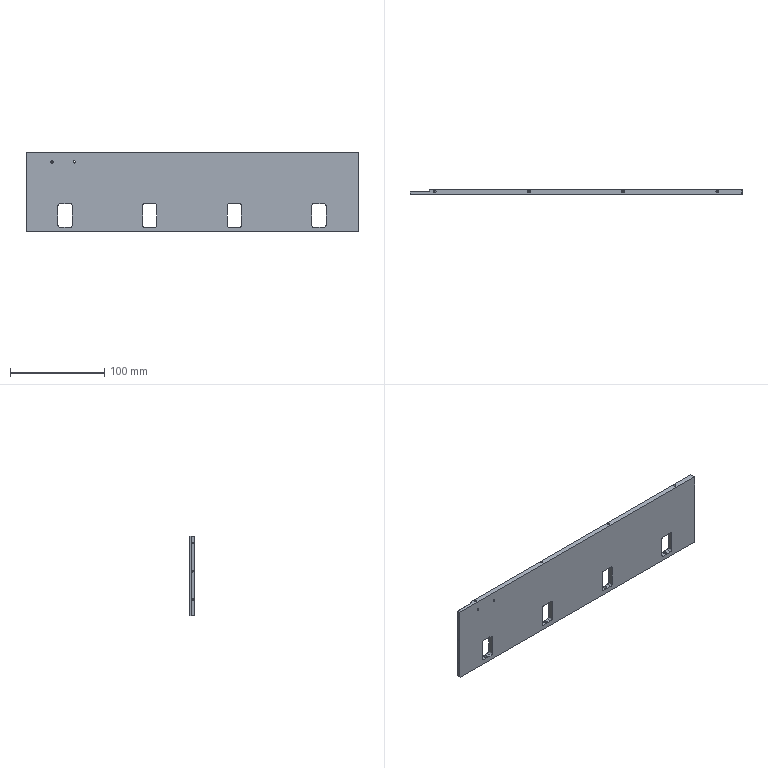CAM job | Mastercam | mm | 9 operations | part box 353 x 5.5 x 85
1. Drill/Counterbore | 2 - 6定位倒角
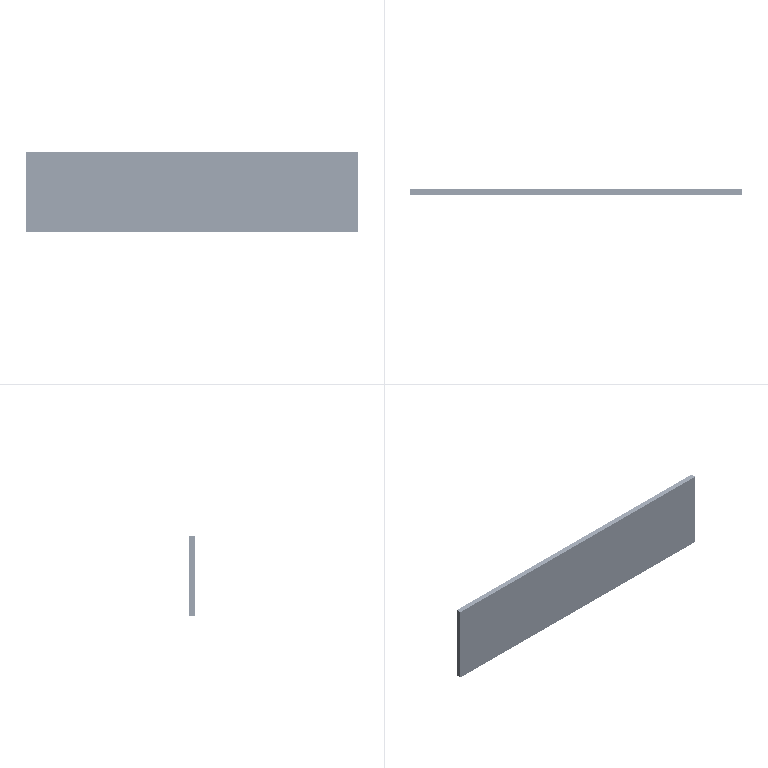2. Peck Drill | 18 - 3.6 钻头
3. Drill/Counterbore | 2 - 6定位倒角
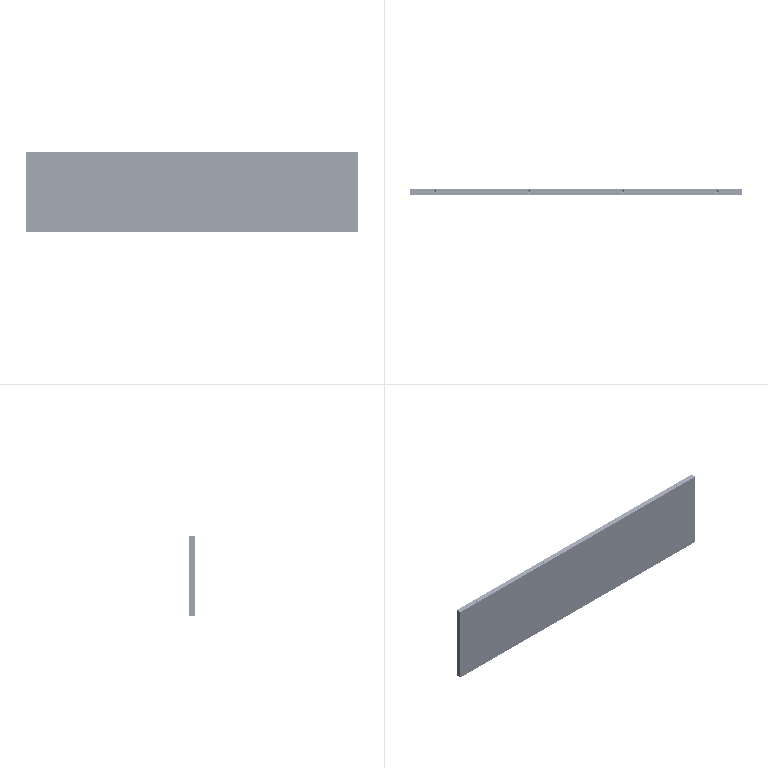4. Peck Drill | 12 - 2.5 钻头
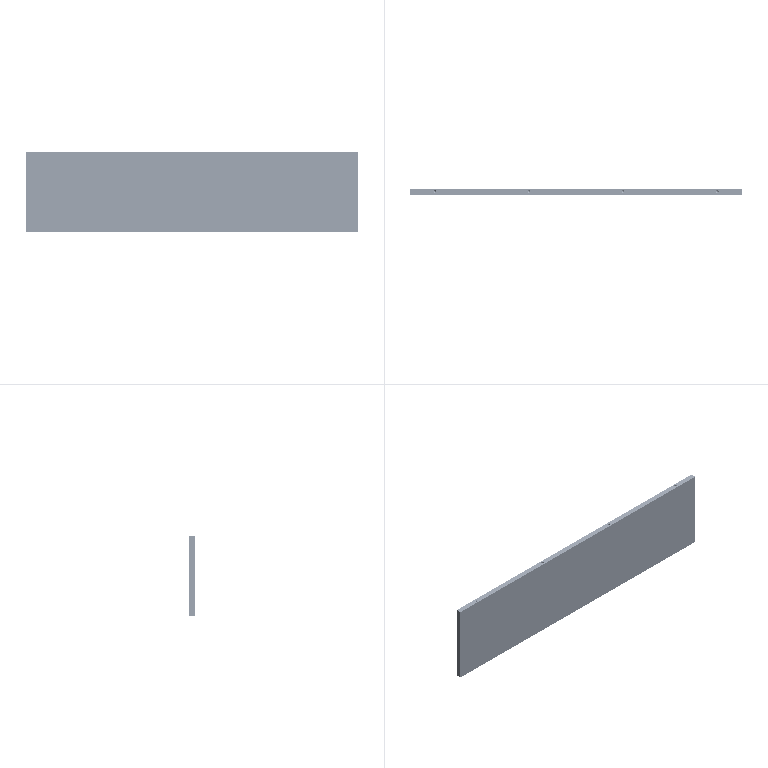5. Peck Drill | 12 - 2.5 钻头
6. Drill/Counterbore | 2 - 6定位倒角
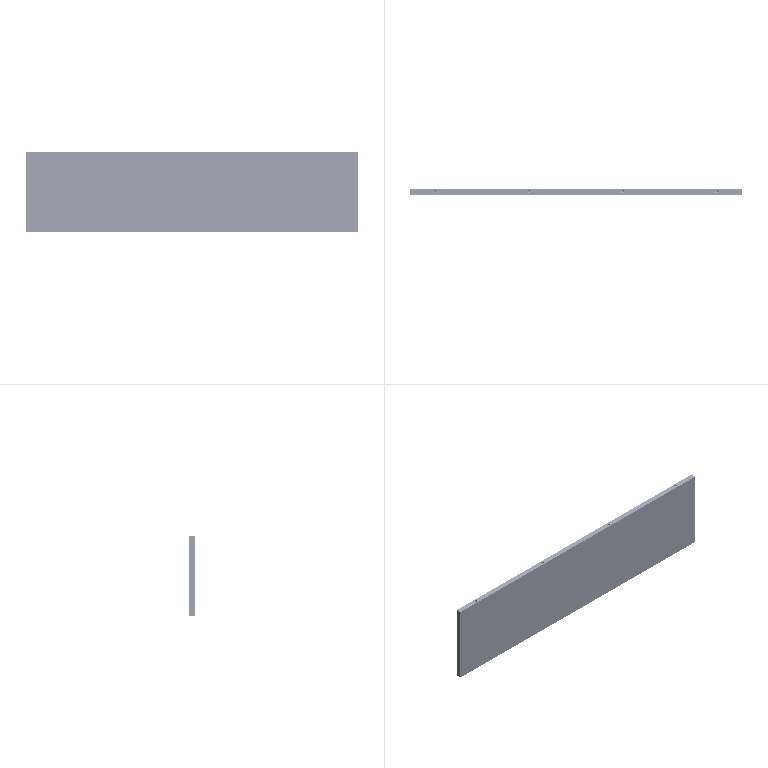7. Peck Drill | 12 - 2.5 钻头
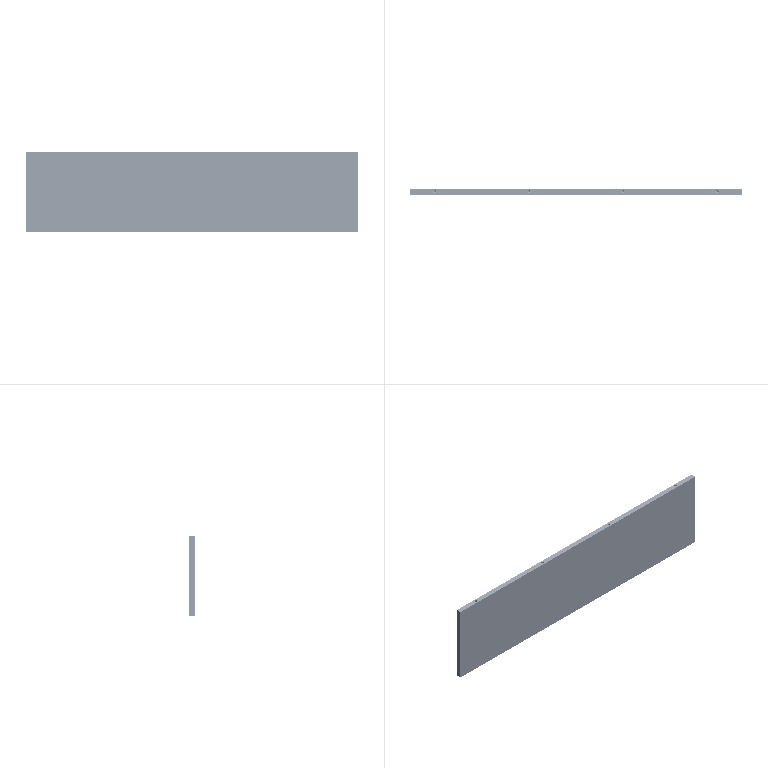8. Drill/Counterbore | 2 - 6定位倒角
9. Peck Drill | 13 - 1.6 钻头